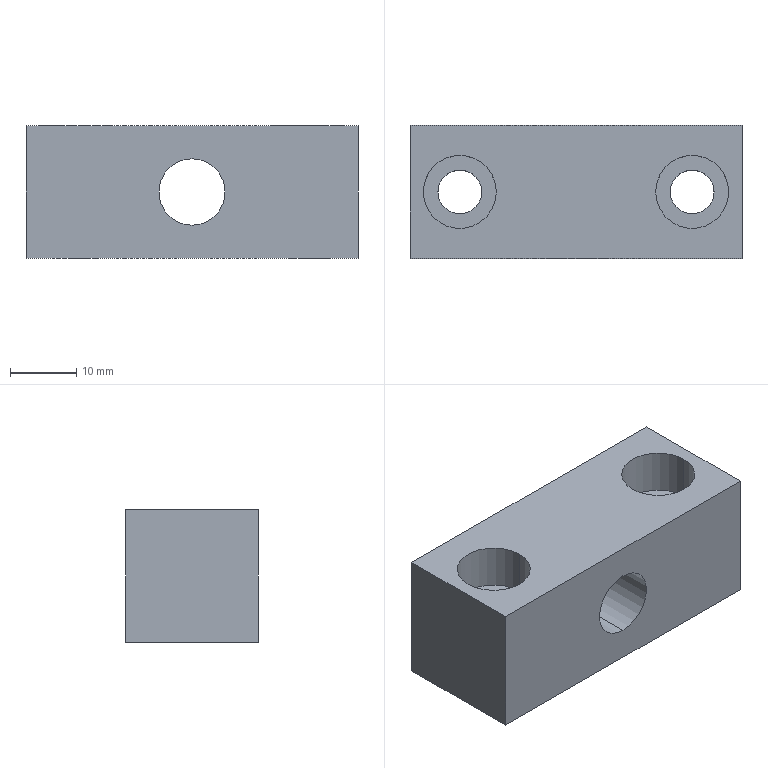Component | SolidWorks | BalanceBlock-0510-2 | 1 solid | 18 faces | box 50 x 20 x 20 mm | volume 16234 mm3 | cylinder 10 | plane 8 | commonest cylinder face diameters 11 x4 6.6 x4 10 x2 | material Q235-A
build123d program:
from build123d import *

# Parameters (mm, degrees)
SKETCH1_W                                          = 50
SKETCH1_H                                          = 20
BOSS_EXTRUDE1_DEPTH                                = 20
HOLE_SIZE_ACCORDING_TO_TYPE_OF_HEX_SOC_D           = 6.6
HOLE_SIZE_ACCORDING_TO_TYPE_OF_HEX_SOC_CBORE_D     = 11
HOLE_SIZE_ACCORDING_TO_TYPE_OF_HEX_SOC_CBORE_DEPTH = 6.8
M10_TAPPED_HOLE1_D                                 = 10


with BuildPart() as part:
    # Sketch1 → Boss-Extrude1 (new body)
    with BuildSketch(Plane.XY):
        Rectangle(SKETCH1_W, SKETCH1_H)
    extrude(amount=BOSS_EXTRUDE1_DEPTH)

    # Hole Size _According to_ Type of Hex Soc (through all)
    with Locations(Plane.XY.offset(20)):
        with Locations((-17.5, 0), (17.5, 0)):
            CounterBoreHole(HOLE_SIZE_ACCORDING_TO_TYPE_OF_HEX_SOC_D / 2, HOLE_SIZE_ACCORDING_TO_TYPE_OF_HEX_SOC_CBORE_D / 2, HOLE_SIZE_ACCORDING_TO_TYPE_OF_HEX_SOC_CBORE_DEPTH)

    # M10 Tapped Hole1 (through all)
    with Locations(Plane(origin=(0, 10, 0), x_dir=(1, 0, 0), z_dir=(0, 1, 0))):
        with Locations((0, -10)):
            Hole(M10_TAPPED_HOLE1_D / 2)


solid = part.part

# Placed as in the assembly
solid = solid.moved(Location((-1407.7, 40.391, 3562.5), (0, 0, 0)))
STEP:
#1=COLOUR_RGB('',0.7922,0.8196,0.9333);
#2=FILL_AREA_STYLE_COLOUR('',#1);
#3=FILL_AREA_STYLE('',(#2));
#4=SURFACE_STYLE_FILL_AREA(#3);
#5=SURFACE_SIDE_STYLE('',(#4));
#6=SURFACE_STYLE_USAGE(.BOTH.,#5);
#7=PRESENTATION_STYLE_ASSIGNMENT((#6));
#8=CARTESIAN_POINT('',(-55.421,1.197,140.453));
#9=VERTEX_POINT('',#8);
#10=CARTESIAN_POINT('',(-55.421,1.197,140.846));
#11=VERTEX_POINT('',#10);
#12=CARTESIAN_POINT('',(-55.421,1.197,140.65));
#13=DIRECTION('',(0.,1.,0.));
#14=DIRECTION('',(0.,0.,1.));
#15=AXIS2_PLACEMENT_3D('',#12,#13,#14);
#16=CIRCLE('',#15,0.1969);
#17=EDGE_CURVE('',#9,#11,#16,.T.);
#18=ORIENTED_EDGE('',*,*,#17,.F.);
#19=CARTESIAN_POINT('',(-55.421,1.984,140.453));
#20=VERTEX_POINT('',#19);
#21=CARTESIAN_POINT('',(-55.421,1.984,140.453));
#22=DIRECTION('',(0.,1.,0.));
#23=VECTOR('',#22,39.37);
#24=LINE('',#21,#23);
#25=EDGE_CURVE('',#9,#20,#24,.T.);
#26=ORIENTED_EDGE('',*,*,#25,.T.);
#27=CARTESIAN_POINT('',(-55.421,1.984,140.846));
#28=VERTEX_POINT('',#27);
#29=CARTESIAN_POINT('',(-55.421,1.984,140.65));
#30=DIRECTION('',(0.,1.,0.));
#31=DIRECTION('',(0.,0.,1.));
#32=AXIS2_PLACEMENT_3D('',#29,#30,#31);
#33=CIRCLE('',#32,0.1969);
#34=EDGE_CURVE('',#20,#28,#33,.T.);
#35=ORIENTED_EDGE('',*,*,#34,.T.);
#36=CARTESIAN_POINT('',(-55.421,1.984,140.846));
#37=DIRECTION('',(0.,1.,0.));
#38=VECTOR('',#37,39.37);
#39=LINE('',#36,#38);
#40=EDGE_CURVE('',#11,#28,#39,.T.);
#41=ORIENTED_EDGE('',*,*,#40,.F.);
#42=EDGE_LOOP('',(#18,#26,#35,#41));
#43=FACE_OUTER_BOUND('',#42,.T.);
#44=CARTESIAN_POINT('',(-55.421,1.984,140.65));
#45=DIRECTION('',(0.,1.,0.));
#46=DIRECTION('',(0.,0.,1.));
#47=AXIS2_PLACEMENT_3D('',#44,#45,#46);
#48=CYLINDRICAL_SURFACE('',#47,0.1969);
#49=ADVANCED_FACE('',(#43),#48,.F.);
#50=CARTESIAN_POINT('',(-56.327,1.59,140.776));
#51=VERTEX_POINT('',#50);
#52=CARTESIAN_POINT('',(-55.894,1.59,140.776));
#53=VERTEX_POINT('',#52);
#54=CARTESIAN_POINT('',(-56.11,1.59,140.776));
#55=DIRECTION('',(0.,0.,1.));
#56=DIRECTION('',(1.,0.,0.));
#57=AXIS2_PLACEMENT_3D('',#54,#55,#56);
#58=CIRCLE('',#57,0.2165);
#59=EDGE_CURVE('',#51,#53,#58,.T.);
#60=ORIENTED_EDGE('',*,*,#59,.F.);
#61=CARTESIAN_POINT('',(-56.327,1.59,141.043));
#62=VERTEX_POINT('',#61);
#63=CARTESIAN_POINT('',(-56.327,1.59,141.043));
#64=DIRECTION('',(0.,0.,1.));
#65=VECTOR('',#64,39.37);
#66=LINE('',#63,#65);
#67=EDGE_CURVE('',#51,#62,#66,.T.);
#68=ORIENTED_EDGE('',*,*,#67,.T.);
#69=CARTESIAN_POINT('',(-55.894,1.59,141.043));
#70=VERTEX_POINT('',#69);
#71=CARTESIAN_POINT('',(-56.11,1.59,141.043));
#72=DIRECTION('',(0.,0.,1.));
#73=DIRECTION('',(1.,0.,0.));
#74=AXIS2_PLACEMENT_3D('',#71,#72,#73);
#75=CIRCLE('',#74,0.2165);
#76=EDGE_CURVE('',#62,#70,#75,.T.);
#77=ORIENTED_EDGE('',*,*,#76,.T.);
#78=CARTESIAN_POINT('',(-55.894,1.59,141.043));
#79=DIRECTION('',(0.,0.,1.));
#80=VECTOR('',#79,39.37);
#81=LINE('',#78,#80);
#82=EDGE_CURVE('',#53,#70,#81,.T.);
#83=ORIENTED_EDGE('',*,*,#82,.F.);
#84=EDGE_LOOP('',(#60,#68,#77,#83));
#85=FACE_OUTER_BOUND('',#84,.T.);
#86=CARTESIAN_POINT('',(-56.11,1.59,141.043));
#87=DIRECTION('',(0.,0.,1.));
#88=DIRECTION('',(1.,0.,0.));
#89=AXIS2_PLACEMENT_3D('',#86,#87,#88);
#90=CYLINDRICAL_SURFACE('',#89,0.2165);
#91=ADVANCED_FACE('',(#85),#90,.F.);
#92=CARTESIAN_POINT('',(-56.24,1.59,140.256));
#93=VERTEX_POINT('',#92);
#94=CARTESIAN_POINT('',(-55.98,1.59,140.256));
#95=VERTEX_POINT('',#94);
#96=CARTESIAN_POINT('',(-56.11,1.59,140.256));
#97=DIRECTION('',(0.,0.,1.));
#98=DIRECTION('',(1.,0.,0.));
#99=AXIS2_PLACEMENT_3D('',#96,#97,#98);
#100=CIRCLE('',#99,0.1299);
#101=EDGE_CURVE('',#93,#95,#100,.T.);
#102=ORIENTED_EDGE('',*,*,#101,.F.);
#103=CARTESIAN_POINT('',(-56.24,1.59,140.776));
#104=VERTEX_POINT('',#103);
#105=CARTESIAN_POINT('',(-56.24,1.59,141.043));
#106=DIRECTION('',(0.,0.,1.));
#107=VECTOR('',#106,39.37);
#108=LINE('',#105,#107);
#109=EDGE_CURVE('',#93,#104,#108,.T.);
#110=ORIENTED_EDGE('',*,*,#109,.T.);
#111=CARTESIAN_POINT('',(-55.98,1.59,140.776));
#112=VERTEX_POINT('',#111);
#113=CARTESIAN_POINT('',(-56.11,1.59,140.776));
#114=DIRECTION('',(0.,0.,1.));
#115=DIRECTION('',(1.,0.,0.));
#116=AXIS2_PLACEMENT_3D('',#113,#114,#115);
#117=CIRCLE('',#116,0.1299);
#118=EDGE_CURVE('',#104,#112,#117,.T.);
#119=ORIENTED_EDGE('',*,*,#118,.T.);
#120=CARTESIAN_POINT('',(-55.98,1.59,141.043));
#121=DIRECTION('',(0.,0.,1.));
#122=VECTOR('',#121,39.37);
#123=LINE('',#120,#122);
#124=EDGE_CURVE('',#95,#112,#123,.T.);
#125=ORIENTED_EDGE('',*,*,#124,.F.);
#126=EDGE_LOOP('',(#102,#110,#119,#125));
#127=FACE_OUTER_BOUND('',#126,.T.);
#128=CARTESIAN_POINT('',(-56.11,1.59,141.043));
#129=DIRECTION('',(0.,0.,1.));
#130=DIRECTION('',(1.,0.,0.));
#131=AXIS2_PLACEMENT_3D('',#128,#129,#130);
#132=CYLINDRICAL_SURFACE('',#131,0.1299);
#133=ADVANCED_FACE('',(#127),#132,.F.);
#134=CARTESIAN_POINT('',(-54.949,1.59,140.776));
#135=VERTEX_POINT('',#134);
#136=CARTESIAN_POINT('',(-54.516,1.59,140.776));
#137=VERTEX_POINT('',#136);
#138=CARTESIAN_POINT('',(-54.732,1.59,140.776));
#139=DIRECTION('',(0.,0.,1.));
#140=DIRECTION('',(1.,0.,0.));
#141=AXIS2_PLACEMENT_3D('',#138,#139,#140);
#142=CIRCLE('',#141,0.2165);
#143=EDGE_CURVE('',#135,#137,#142,.T.);
#144=ORIENTED_EDGE('',*,*,#143,.F.);
#145=CARTESIAN_POINT('',(-54.949,1.59,141.043));
#146=VERTEX_POINT('',#145);
#147=CARTESIAN_POINT('',(-54.949,1.59,141.043));
#148=DIRECTION('',(0.,0.,1.));
#149=VECTOR('',#148,39.37);
#150=LINE('',#147,#149);
#151=EDGE_CURVE('',#135,#146,#150,.T.);
#152=ORIENTED_EDGE('',*,*,#151,.T.);
#153=CARTESIAN_POINT('',(-54.516,1.59,141.043));
#154=VERTEX_POINT('',#153);
#155=CARTESIAN_POINT('',(-54.732,1.59,141.043));
#156=DIRECTION('',(0.,0.,1.));
#157=DIRECTION('',(1.,0.,0.));
#158=AXIS2_PLACEMENT_3D('',#155,#156,#157);
#159=CIRCLE('',#158,0.2165);
#160=EDGE_CURVE('',#146,#154,#159,.T.);
#161=ORIENTED_EDGE('',*,*,#160,.T.);
#162=CARTESIAN_POINT('',(-54.516,1.59,141.043));
#163=DIRECTION('',(0.,0.,1.));
#164=VECTOR('',#163,39.37);
#165=LINE('',#162,#164);
#166=EDGE_CURVE('',#137,#154,#165,.T.);
#167=ORIENTED_EDGE('',*,*,#166,.F.);
#168=EDGE_LOOP('',(#144,#152,#161,#167));
#169=FACE_OUTER_BOUND('',#168,.T.);
#170=CARTESIAN_POINT('',(-54.732,1.59,141.043));
#171=DIRECTION('',(0.,0.,1.));
#172=DIRECTION('',(1.,0.,0.));
#173=AXIS2_PLACEMENT_3D('',#170,#171,#172);
#174=CYLINDRICAL_SURFACE('',#173,0.2165);
#175=ADVANCED_FACE('',(#169),#174,.F.);
#176=CARTESIAN_POINT('',(-54.862,1.59,140.256));
#177=VERTEX_POINT('',#176);
#178=CARTESIAN_POINT('',(-54.602,1.59,140.256));
#179=VERTEX_POINT('',#178);
#180=CARTESIAN_POINT('',(-54.732,1.59,140.256));
#181=DIRECTION('',(0.,0.,1.));
#182=DIRECTION('',(1.,0.,0.));
#183=AXIS2_PLACEMENT_3D('',#180,#181,#182);
#184=CIRCLE('',#183,0.1299);
#185=EDGE_CURVE('',#177,#179,#184,.T.);
#186=ORIENTED_EDGE('',*,*,#185,.F.);
#187=CARTESIAN_POINT('',(-54.862,1.59,140.776));
#188=VERTEX_POINT('',#187);
#189=CARTESIAN_POINT('',(-54.862,1.59,141.043));
#190=DIRECTION('',(0.,0.,1.));
#191=VECTOR('',#190,39.37);
#192=LINE('',#189,#191);
#193=EDGE_CURVE('',#177,#188,#192,.T.);
#194=ORIENTED_EDGE('',*,*,#193,.T.);
#195=CARTESIAN_POINT('',(-54.602,1.59,140.776));
#196=VERTEX_POINT('',#195);
#197=CARTESIAN_POINT('',(-54.732,1.59,140.776));
#198=DIRECTION('',(0.,0.,1.));
#199=DIRECTION('',(1.,0.,0.));
#200=AXIS2_PLACEMENT_3D('',#197,#198,#199);
#201=CIRCLE('',#200,0.1299);
#202=EDGE_CURVE('',#188,#196,#201,.T.);
#203=ORIENTED_EDGE('',*,*,#202,.T.);
#204=CARTESIAN_POINT('',(-54.602,1.59,141.043));
#205=DIRECTION('',(0.,0.,1.));
#206=VECTOR('',#205,39.37);
#207=LINE('',#204,#206);
#208=EDGE_CURVE('',#179,#196,#207,.T.);
#209=ORIENTED_EDGE('',*,*,#208,.F.);
#210=EDGE_LOOP('',(#186,#194,#203,#209));
#211=FACE_OUTER_BOUND('',#210,.T.);
#212=CARTESIAN_POINT('',(-54.732,1.59,141.043));
#213=DIRECTION('',(0.,0.,1.));
#214=DIRECTION('',(1.,0.,0.));
#215=AXIS2_PLACEMENT_3D('',#212,#213,#214);
#216=CYLINDRICAL_SURFACE('',#215,0.1299);
#217=ADVANCED_FACE('',(#211),#216,.F.);
#218=CARTESIAN_POINT('',(-54.437,1.197,140.256));
#219=VERTEX_POINT('',#218);
#220=CARTESIAN_POINT('',(-54.437,1.984,140.256));
#221=VERTEX_POINT('',#220);
#222=CARTESIAN_POINT('',(-54.437,1.984,140.256));
#223=DIRECTION('',(0.,1.,0.));
#224=VECTOR('',#223,39.37);
#225=LINE('',#222,#224);
#226=EDGE_CURVE('',#219,#221,#225,.T.);
#227=ORIENTED_EDGE('',*,*,#226,.T.);
#228=CARTESIAN_POINT('',(-54.437,1.984,141.043));
#229=VERTEX_POINT('',#228);
#230=CARTESIAN_POINT('',(-54.437,1.984,141.043));
#231=DIRECTION('',(0.,0.,-1.));
#232=VECTOR('',#231,39.37);
#233=LINE('',#230,#232);
#234=EDGE_CURVE('',#229,#221,#233,.T.);
#235=ORIENTED_EDGE('',*,*,#234,.F.);
#236=CARTESIAN_POINT('',(-54.437,1.197,141.043));
#237=VERTEX_POINT('',#236);
#238=CARTESIAN_POINT('',(-54.437,1.984,141.043));
#239=DIRECTION('',(0.,1.,0.));
#240=VECTOR('',#239,39.37);
#241=LINE('',#238,#240);
#242=EDGE_CURVE('',#237,#229,#241,.T.);
#243=ORIENTED_EDGE('',*,*,#242,.F.);
#244=CARTESIAN_POINT('',(-54.437,1.197,141.043));
#245=DIRECTION('',(0.,0.,-1.));
#246=VECTOR('',#245,39.37);
#247=LINE('',#244,#246);
#248=EDGE_CURVE('',#237,#219,#247,.T.);
#249=ORIENTED_EDGE('',*,*,#248,.T.);
#250=EDGE_LOOP('',(#227,#235,#243,#249));
#251=FACE_OUTER_BOUND('',#250,.T.);
#252=CARTESIAN_POINT('',(-54.437,1.984,141.043));
#253=DIRECTION('',(-1.,0.,0.));
#254=DIRECTION('',(0.,0.,1.));
#255=AXIS2_PLACEMENT_3D('',#252,#253,#254);
#256=PLANE('',#255);
#257=ADVANCED_FACE('',(#251),#256,.F.);
#258=CARTESIAN_POINT('',(-55.421,1.984,140.65));
#259=DIRECTION('',(0.,1.,0.));
#260=DIRECTION('',(0.,0.,1.));
#261=AXIS2_PLACEMENT_3D('',#258,#259,#260);
#262=CIRCLE('',#261,0.1969);
#263=EDGE_CURVE('',#28,#20,#262,.T.);
#264=ORIENTED_EDGE('',*,*,#263,.F.);
#265=ORIENTED_EDGE('',*,*,#34,.F.);
#266=EDGE_LOOP('',(#264,#265));
#267=FACE_BOUND('',#266,.T.);
#268=CARTESIAN_POINT('',(-56.406,1.984,140.256));
#269=VERTEX_POINT('',#268);
#270=CARTESIAN_POINT('',(-56.406,1.984,140.256));
#271=DIRECTION('',(-1.,0.,0.));
#272=VECTOR('',#271,39.37);
#273=LINE('',#270,#272);
#274=EDGE_CURVE('',#221,#269,#273,.T.);
#275=ORIENTED_EDGE('',*,*,#274,.T.);
#276=CARTESIAN_POINT('',(-56.406,1.984,141.043));
#277=VERTEX_POINT('',#276);
#278=CARTESIAN_POINT('',(-56.406,1.984,141.043));
#279=DIRECTION('',(0.,0.,-1.));
#280=VECTOR('',#279,39.37);
#281=LINE('',#278,#280);
#282=EDGE_CURVE('',#277,#269,#281,.T.);
#283=ORIENTED_EDGE('',*,*,#282,.F.);
#284=CARTESIAN_POINT('',(-56.406,1.984,141.043));
#285=DIRECTION('',(-1.,0.,0.));
#286=VECTOR('',#285,39.37);
#287=LINE('',#284,#286);
#288=EDGE_CURVE('',#229,#277,#287,.T.);
#289=ORIENTED_EDGE('',*,*,#288,.F.);
#290=ORIENTED_EDGE('',*,*,#234,.T.);
#291=EDGE_LOOP('',(#275,#283,#289,#290));
#292=FACE_OUTER_BOUND('',#291,.T.);
#293=CARTESIAN_POINT('',(-56.406,1.984,141.043));
#294=DIRECTION('',(0.,-1.,0.));
#295=DIRECTION('',(0.,0.,-1.));
#296=AXIS2_PLACEMENT_3D('',#293,#294,#295);
#297=PLANE('',#296);
#298=ADVANCED_FACE('',(#267,#292),#297,.F.);
#299=CARTESIAN_POINT('',(-56.406,1.197,140.256));
#300=VERTEX_POINT('',#299);
#301=CARTESIAN_POINT('',(-56.406,1.984,140.256));
#302=DIRECTION('',(0.,-1.,0.));
#303=VECTOR('',#302,39.37);
#304=LINE('',#301,#303);
#305=EDGE_CURVE('',#269,#300,#304,.T.);
#306=ORIENTED_EDGE('',*,*,#305,.T.);
#307=CARTESIAN_POINT('',(-56.406,1.197,141.043));
#308=VERTEX_POINT('',#307);
#309=CARTESIAN_POINT('',(-56.406,1.197,141.043));
#310=DIRECTION('',(0.,0.,-1.));
#311=VECTOR('',#310,39.37);
#312=LINE('',#309,#311);
#313=EDGE_CURVE('',#308,#300,#312,.T.);
#314=ORIENTED_EDGE('',*,*,#313,.F.);
#315=CARTESIAN_POINT('',(-56.406,1.984,141.043));
#316=DIRECTION('',(0.,-1.,0.));
#317=VECTOR('',#316,39.37);
#318=LINE('',#315,#317);
#319=EDGE_CURVE('',#277,#308,#318,.T.);
#320=ORIENTED_EDGE('',*,*,#319,.F.);
#321=ORIENTED_EDGE('',*,*,#282,.T.);
#322=EDGE_LOOP('',(#306,#314,#320,#321));
#323=FACE_OUTER_BOUND('',#322,.T.);
#324=CARTESIAN_POINT('',(-56.406,1.984,141.043));
#325=DIRECTION('',(1.,0.,0.));
#326=DIRECTION('',(0.,0.,-1.));
#327=AXIS2_PLACEMENT_3D('',#324,#325,#326);
#328=PLANE('',#327);
#329=ADVANCED_FACE('',(#323),#328,.F.);
#330=CARTESIAN_POINT('',(-55.421,1.197,140.65));
#331=DIRECTION('',(0.,1.,0.));
#332=DIRECTION('',(0.,0.,1.));
#333=AXIS2_PLACEMENT_3D('',#330,#331,#332);
#334=CIRCLE('',#333,0.1969);
#335=EDGE_CURVE('',#11,#9,#334,.T.);
#336=ORIENTED_EDGE('',*,*,#335,.T.);
#337=ORIENTED_EDGE('',*,*,#17,.T.);
#338=EDGE_LOOP('',(#336,#337));
#339=FACE_BOUND('',#338,.T.);
#340=CARTESIAN_POINT('',(-56.406,1.197,140.256));
#341=DIRECTION('',(1.,0.,0.));
#342=VECTOR('',#341,39.37);
#343=LINE('',#340,#342);
#344=EDGE_CURVE('',#300,#219,#343,.T.);
#345=ORIENTED_EDGE('',*,*,#344,.T.);
#346=ORIENTED_EDGE('',*,*,#248,.F.);
#347=CARTESIAN_POINT('',(-56.406,1.197,141.043));
#348=DIRECTION('',(1.,0.,0.));
#349=VECTOR('',#348,39.37);
#350=LINE('',#347,#349);
#351=EDGE_CURVE('',#308,#237,#350,.T.);
#352=ORIENTED_EDGE('',*,*,#351,.F.);
#353=ORIENTED_EDGE('',*,*,#313,.T.);
#354=EDGE_LOOP('',(#345,#346,#352,#353));
#355=FACE_OUTER_BOUND('',#354,.T.);
#356=CARTESIAN_POINT('',(-56.406,1.197,141.043));
#357=DIRECTION('',(0.,1.,0.));
#358=DIRECTION('',(0.,0.,1.));
#359=AXIS2_PLACEMENT_3D('',#356,#357,#358);
#360=PLANE('',#359);
#361=ADVANCED_FACE('',(#339,#355),#360,.F.);
#362=CARTESIAN_POINT('',(-56.11,1.59,141.043));
#363=DIRECTION('',(0.,0.,1.));
#364=DIRECTION('',(1.,0.,0.));
#365=AXIS2_PLACEMENT_3D('',#362,#363,#364);
#366=CIRCLE('',#365,0.2165);
#367=EDGE_CURVE('',#70,#62,#366,.T.);
#368=ORIENTED_EDGE('',*,*,#367,.F.);
#369=ORIENTED_EDGE('',*,*,#76,.F.);
#370=EDGE_LOOP('',(#368,#369));
#371=FACE_BOUND('',#370,.T.);
#372=CARTESIAN_POINT('',(-54.732,1.59,141.043));
#373=DIRECTION('',(0.,0.,1.));
#374=DIRECTION('',(1.,0.,0.));
#375=AXIS2_PLACEMENT_3D('',#372,#373,#374);
#376=CIRCLE('',#375,0.2165);
#377=EDGE_CURVE('',#154,#146,#376,.T.);
#378=ORIENTED_EDGE('',*,*,#377,.F.);
#379=ORIENTED_EDGE('',*,*,#160,.F.);
#380=EDGE_LOOP('',(#378,#379));
#381=FACE_BOUND('',#380,.T.);
#382=ORIENTED_EDGE('',*,*,#242,.T.);
#383=ORIENTED_EDGE('',*,*,#288,.T.);
#384=ORIENTED_EDGE('',*,*,#319,.T.);
#385=ORIENTED_EDGE('',*,*,#351,.T.);
#386=EDGE_LOOP('',(#382,#383,#384,#385));
#387=FACE_OUTER_BOUND('',#386,.T.);
#388=CARTESIAN_POINT('',(-55.421,1.59,141.043));
#389=DIRECTION('',(0.,0.,1.));
#390=DIRECTION('',(1.,0.,0.));
#391=AXIS2_PLACEMENT_3D('',#388,#389,#390);
#392=PLANE('',#391);
#393=ADVANCED_FACE('',(#371,#381,#387),#392,.T.);
#394=CARTESIAN_POINT('',(-56.11,1.59,140.256));
#395=DIRECTION('',(0.,0.,1.));
#396=DIRECTION('',(1.,0.,0.));
#397=AXIS2_PLACEMENT_3D('',#394,#395,#396);
#398=CIRCLE('',#397,0.1299);
#399=EDGE_CURVE('',#95,#93,#398,.T.);
#400=ORIENTED_EDGE('',*,*,#399,.T.);
#401=ORIENTED_EDGE('',*,*,#101,.T.);
#402=EDGE_LOOP('',(#400,#401));
#403=FACE_BOUND('',#402,.T.);
#404=CARTESIAN_POINT('',(-54.732,1.59,140.256));
#405=DIRECTION('',(0.,0.,1.));
#406=DIRECTION('',(1.,0.,0.));
#407=AXIS2_PLACEMENT_3D('',#404,#405,#406);
#408=CIRCLE('',#407,0.1299);
#409=EDGE_CURVE('',#179,#177,#408,.T.);
#410=ORIENTED_EDGE('',*,*,#409,.T.);
#411=ORIENTED_EDGE('',*,*,#185,.T.);
#412=EDGE_LOOP('',(#410,#411));
#413=FACE_BOUND('',#412,.T.);
#414=ORIENTED_EDGE('',*,*,#226,.F.);
#415=ORIENTED_EDGE('',*,*,#344,.F.);
#416=ORIENTED_EDGE('',*,*,#305,.F.);
#417=ORIENTED_EDGE('',*,*,#274,.F.);
#418=EDGE_LOOP('',(#414,#415,#416,#417));
#419=FACE_OUTER_BOUND('',#418,.T.);
#420=CARTESIAN_POINT('',(-55.421,1.59,140.256));
#421=DIRECTION('',(0.,0.,1.));
#422=DIRECTION('',(1.,0.,0.));
#423=AXIS2_PLACEMENT_3D('',#420,#421,#422);
#424=PLANE('',#423);
#425=ADVANCED_FACE('',(#403,#413,#419),#424,.F.);
#426=ORIENTED_EDGE('',*,*,#193,.F.);
#427=ORIENTED_EDGE('',*,*,#409,.F.);
#428=ORIENTED_EDGE('',*,*,#208,.T.);
#429=CARTESIAN_POINT('',(-54.732,1.59,140.776));
#430=DIRECTION('',(0.,0.,1.));
#431=DIRECTION('',(1.,0.,0.));
#432=AXIS2_PLACEMENT_3D('',#429,#430,#431);
#433=CIRCLE('',#432,0.1299);
#434=EDGE_CURVE('',#196,#188,#433,.T.);
#435=ORIENTED_EDGE('',*,*,#434,.T.);
#436=EDGE_LOOP('',(#426,#427,#428,#435));
#437=FACE_OUTER_BOUND('',#436,.T.);
#438=CARTESIAN_POINT('',(-54.732,1.59,141.043));
#439=DIRECTION('',(0.,0.,1.));
#440=DIRECTION('',(1.,0.,0.));
#441=AXIS2_PLACEMENT_3D('',#438,#439,#440);
#442=CYLINDRICAL_SURFACE('',#441,0.1299);
#443=ADVANCED_FACE('',(#437),#442,.F.);
#444=ORIENTED_EDGE('',*,*,#434,.F.);
#445=ORIENTED_EDGE('',*,*,#202,.F.);
#446=EDGE_LOOP('',(#444,#445));
#447=FACE_BOUND('',#446,.T.);
#448=CARTESIAN_POINT('',(-54.732,1.59,140.776));
#449=DIRECTION('',(0.,0.,1.));
#450=DIRECTION('',(1.,0.,0.));
#451=AXIS2_PLACEMENT_3D('',#448,#449,#450);
#452=CIRCLE('',#451,0.2165);
#453=EDGE_CURVE('',#137,#135,#452,.T.);
#454=ORIENTED_EDGE('',*,*,#453,.T.);
#455=ORIENTED_EDGE('',*,*,#143,.T.);
#456=EDGE_LOOP('',(#454,#455));
#457=FACE_OUTER_BOUND('',#456,.T.);
#458=CARTESIAN_POINT('',(-54.602,1.59,140.776));
#459=DIRECTION('',(0.,0.,-1.));
#460=DIRECTION('',(-1.,0.,0.));
#461=AXIS2_PLACEMENT_3D('',#458,#459,#460);
#462=PLANE('',#461);
#463=ADVANCED_FACE('',(#447,#457),#462,.F.);
#464=ORIENTED_EDGE('',*,*,#151,.F.);
#465=ORIENTED_EDGE('',*,*,#453,.F.);
#466=ORIENTED_EDGE('',*,*,#166,.T.);
#467=ORIENTED_EDGE('',*,*,#377,.T.);
#468=EDGE_LOOP('',(#464,#465,#466,#467));
#469=FACE_OUTER_BOUND('',#468,.T.);
#470=CARTESIAN_POINT('',(-54.732,1.59,141.043));
#471=DIRECTION('',(0.,0.,1.));
#472=DIRECTION('',(1.,0.,0.));
#473=AXIS2_PLACEMENT_3D('',#470,#471,#472);
#474=CYLINDRICAL_SURFACE('',#473,0.2165);
#475=ADVANCED_FACE('',(#469),#474,.F.);
#476=ORIENTED_EDGE('',*,*,#109,.F.);
#477=ORIENTED_EDGE('',*,*,#399,.F.);
#478=ORIENTED_EDGE('',*,*,#124,.T.);
#479=CARTESIAN_POINT('',(-56.11,1.59,140.776));
#480=DIRECTION('',(0.,0.,1.));
#481=DIRECTION('',(1.,0.,0.));
#482=AXIS2_PLACEMENT_3D('',#479,#480,#481);
#483=CIRCLE('',#482,0.1299);
#484=EDGE_CURVE('',#112,#104,#483,.T.);
#485=ORIENTED_EDGE('',*,*,#484,.T.);
#486=EDGE_LOOP('',(#476,#477,#478,#485));
#487=FACE_OUTER_BOUND('',#486,.T.);
#488=CARTESIAN_POINT('',(-56.11,1.59,141.043));
#489=DIRECTION('',(0.,0.,1.));
#490=DIRECTION('',(1.,0.,0.));
#491=AXIS2_PLACEMENT_3D('',#488,#489,#490);
#492=CYLINDRICAL_SURFACE('',#491,0.1299);
#493=ADVANCED_FACE('',(#487),#492,.F.);
#494=ORIENTED_EDGE('',*,*,#484,.F.);
#495=ORIENTED_EDGE('',*,*,#118,.F.);
#496=EDGE_LOOP('',(#494,#495));
#497=FACE_BOUND('',#496,.T.);
#498=CARTESIAN_POINT('',(-56.11,1.59,140.776));
#499=DIRECTION('',(0.,0.,1.));
#500=DIRECTION('',(1.,0.,0.));
#501=AXIS2_PLACEMENT_3D('',#498,#499,#500);
#502=CIRCLE('',#501,0.2165);
#503=EDGE_CURVE('',#53,#51,#502,.T.);
#504=ORIENTED_EDGE('',*,*,#503,.T.);
#505=ORIENTED_EDGE('',*,*,#59,.T.);
#506=EDGE_LOOP('',(#504,#505));
#507=FACE_OUTER_BOUND('',#506,.T.);
#508=CARTESIAN_POINT('',(-55.98,1.59,140.776));
#509=DIRECTION('',(0.,0.,-1.));
#510=DIRECTION('',(-1.,0.,0.));
#511=AXIS2_PLACEMENT_3D('',#508,#509,#510);
#512=PLANE('',#511);
#513=ADVANCED_FACE('',(#497,#507),#512,.F.);
#514=ORIENTED_EDGE('',*,*,#67,.F.);
#515=ORIENTED_EDGE('',*,*,#503,.F.);
#516=ORIENTED_EDGE('',*,*,#82,.T.);
#517=ORIENTED_EDGE('',*,*,#367,.T.);
#518=EDGE_LOOP('',(#514,#515,#516,#517));
#519=FACE_OUTER_BOUND('',#518,.T.);
#520=CARTESIAN_POINT('',(-56.11,1.59,141.043));
#521=DIRECTION('',(0.,0.,1.));
#522=DIRECTION('',(1.,0.,0.));
#523=AXIS2_PLACEMENT_3D('',#520,#521,#522);
#524=CYLINDRICAL_SURFACE('',#523,0.2165);
#525=ADVANCED_FACE('',(#519),#524,.F.);
#526=ORIENTED_EDGE('',*,*,#25,.F.);
#527=ORIENTED_EDGE('',*,*,#335,.F.);
#528=ORIENTED_EDGE('',*,*,#40,.T.);
#529=ORIENTED_EDGE('',*,*,#263,.T.);
#530=EDGE_LOOP('',(#526,#527,#528,#529));
#531=FACE_OUTER_BOUND('',#530,.T.);
#532=CARTESIAN_POINT('',(-55.421,1.984,140.65));
#533=DIRECTION('',(0.,1.,0.));
#534=DIRECTION('',(0.,0.,1.));
#535=AXIS2_PLACEMENT_3D('',#532,#533,#534);
#536=CYLINDRICAL_SURFACE('',#535,0.1969);
#537=ADVANCED_FACE('',(#531),#536,.F.);
#538=CLOSED_SHELL('',(#49,#91,#133,#175,#217,#257,#298,#329,#361,#393,#425,#443,#463,#475,#493,#513,#525,#537));
#539=MANIFOLD_SOLID_BREP('',#538);
#540=STYLED_ITEM('',(#7),#539);
#541=PRESENTATION_LAYER_ASSIGNMENT('','',(#540));
#542=(LENGTH_UNIT()NAMED_UNIT(*)SI_UNIT($,.METRE.));
#543=LENGTH_MEASURE_WITH_UNIT(LENGTH_MEASURE(0.0254),#542);
#544=DIMENSIONAL_EXPONENTS(1.,0.,0.,0.,0.,0.,0.);
#545=(CONVERSION_BASED_UNIT('',#543)LENGTH_UNIT()NAMED_UNIT(#544));
#546=UNCERTAINTY_MEASURE_WITH_UNIT(LENGTH_MEASURE(0.00001),#545,'','');
#547=(NAMED_UNIT(*)PLANE_ANGLE_UNIT()SI_UNIT($,.RADIAN.));
#548=(NAMED_UNIT(*)SI_UNIT($,.STERADIAN.)SOLID_ANGLE_UNIT());
#549=(GEOMETRIC_REPRESENTATION_CONTEXT(3)GLOBAL_UNCERTAINTY_ASSIGNED_CONTEXT((#546))GLOBAL_UNIT_ASSIGNED_CONTEXT((#545,#547,#548))REPRESENTATION_CONTEXT('',''));
#550=MECHANICAL_DESIGN_GEOMETRIC_PRESENTATION_REPRESENTATION('',(#540),#549);
#551=CARTESIAN_POINT('',(0.,0.,0.));
#552=DIRECTION('',(0.,0.,1.));
#553=DIRECTION('',(1.,0.,0.));
#554=AXIS2_PLACEMENT_3D('',#551,#552,#553);
#555=(LENGTH_UNIT()NAMED_UNIT(*)SI_UNIT($,.METRE.));
#556=LENGTH_MEASURE_WITH_UNIT(LENGTH_MEASURE(0.0254),#555);
#557=DIMENSIONAL_EXPONENTS(1.,0.,0.,0.,0.,0.,0.);
#558=(CONVERSION_BASED_UNIT('',#556)LENGTH_UNIT()NAMED_UNIT(#557));
#559=UNCERTAINTY_MEASURE_WITH_UNIT(LENGTH_MEASURE(0.00001),#558,'','');
#560=(NAMED_UNIT(*)PLANE_ANGLE_UNIT()SI_UNIT($,.RADIAN.));
#561=(NAMED_UNIT(*)SI_UNIT($,.STERADIAN.)SOLID_ANGLE_UNIT());
#562=(GEOMETRIC_REPRESENTATION_CONTEXT(3)GLOBAL_UNCERTAINTY_ASSIGNED_CONTEXT((#559))GLOBAL_UNIT_ASSIGNED_CONTEXT((#558,#560,#561))REPRESENTATION_CONTEXT('',''));
#563=ADVANCED_BREP_SHAPE_REPRESENTATION('',(#539,#554),#562);